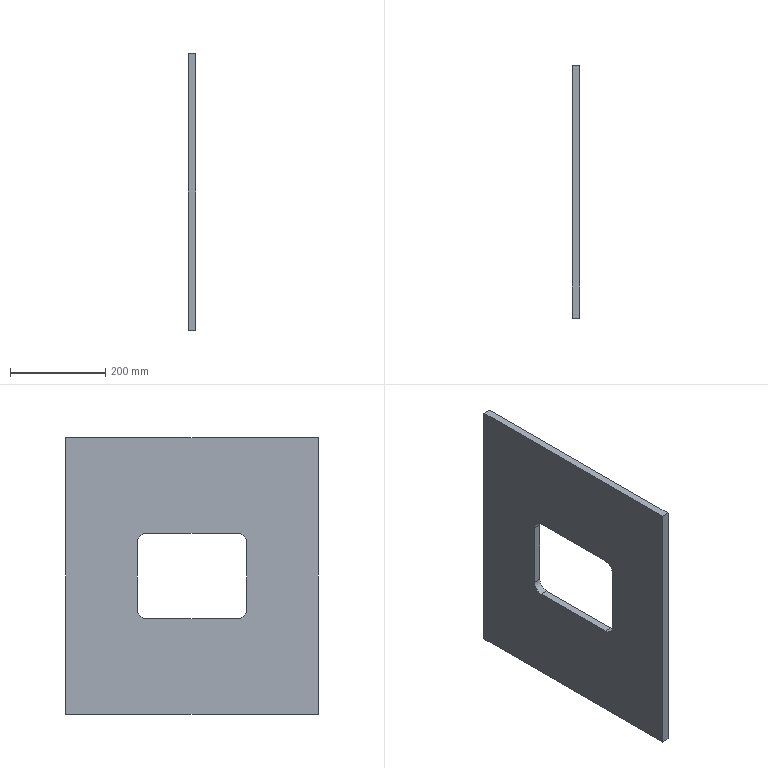Component | SolidWorks | ElectromagneticBeamRibPlate3-2 | 1 solid | 14 faces | box 16 x 530 x 580 mm | volume 4261494 mm3 | plane 10 | cylinder 4 | commonest cylinder face diameters 40 x4 | material Plain Carbon Steel
STEP:
#1=COLOUR_RGB('',0.7922,0.8196,0.9333);
#2=FILL_AREA_STYLE_COLOUR('',#1);
#3=FILL_AREA_STYLE('',(#2));
#4=SURFACE_STYLE_FILL_AREA(#3);
#5=SURFACE_SIDE_STYLE('',(#4));
#6=SURFACE_STYLE_USAGE(.BOTH.,#5);
#7=PRESENTATION_STYLE_ASSIGNMENT((#6));
#8=CARTESIAN_POINT('',(417.423,116.997,262.758));
#9=VERTEX_POINT('',#8);
#10=CARTESIAN_POINT('',(417.423,116.997,239.923));
#11=VERTEX_POINT('',#10);
#12=CARTESIAN_POINT('',(417.423,116.997,262.758));
#13=DIRECTION('',(0.,0.,-1.));
#14=VECTOR('',#13,39.37);
#15=LINE('',#12,#14);
#16=EDGE_CURVE('',#9,#11,#15,.T.);
#17=ORIENTED_EDGE('',*,*,#16,.F.);
#18=CARTESIAN_POINT('',(416.793,116.997,262.758));
#19=VERTEX_POINT('',#18);
#20=CARTESIAN_POINT('',(416.793,116.997,262.758));
#21=DIRECTION('',(1.,-0.,0.));
#22=VECTOR('',#21,39.37);
#23=LINE('',#20,#22);
#24=EDGE_CURVE('',#19,#9,#23,.T.);
#25=ORIENTED_EDGE('',*,*,#24,.F.);
#26=CARTESIAN_POINT('',(416.793,116.997,239.923));
#27=VERTEX_POINT('',#26);
#28=CARTESIAN_POINT('',(416.793,116.997,262.758));
#29=DIRECTION('',(0.,0.,-1.));
#30=VECTOR('',#29,39.37);
#31=LINE('',#28,#30);
#32=EDGE_CURVE('',#19,#27,#31,.T.);
#33=ORIENTED_EDGE('',*,*,#32,.T.);
#34=CARTESIAN_POINT('',(416.793,116.997,239.923));
#35=DIRECTION('',(1.,-0.,0.));
#36=VECTOR('',#35,39.37);
#37=LINE('',#34,#36);
#38=EDGE_CURVE('',#27,#11,#37,.T.);
#39=ORIENTED_EDGE('',*,*,#38,.T.);
#40=EDGE_LOOP('',(#17,#25,#33,#39));
#41=FACE_OUTER_BOUND('',#40,.T.);
#42=CARTESIAN_POINT('',(416.793,116.997,262.758));
#43=DIRECTION('',(-0.,-1.,-0.));
#44=DIRECTION('',(0.,0.,-1.));
#45=AXIS2_PLACEMENT_3D('',#42,#43,#44);
#46=PLANE('',#45);
#47=ADVANCED_FACE('',(#41),#46,.T.);
#48=CARTESIAN_POINT('',(417.423,137.863,262.758));
#49=VERTEX_POINT('',#48);
#50=CARTESIAN_POINT('',(417.423,116.997,262.758));
#51=DIRECTION('',(-0.,-1.,0.));
#52=VECTOR('',#51,39.37);
#53=LINE('',#50,#52);
#54=EDGE_CURVE('',#49,#9,#53,.T.);
#55=ORIENTED_EDGE('',*,*,#54,.F.);
#56=CARTESIAN_POINT('',(416.793,137.863,262.758));
#57=VERTEX_POINT('',#56);
#58=CARTESIAN_POINT('',(416.793,137.863,262.758));
#59=DIRECTION('',(1.,-0.,0.));
#60=VECTOR('',#59,39.37);
#61=LINE('',#58,#60);
#62=EDGE_CURVE('',#57,#49,#61,.T.);
#63=ORIENTED_EDGE('',*,*,#62,.F.);
#64=CARTESIAN_POINT('',(416.793,116.997,262.758));
#65=DIRECTION('',(-0.,-1.,0.));
#66=VECTOR('',#65,39.37);
#67=LINE('',#64,#66);
#68=EDGE_CURVE('',#57,#19,#67,.T.);
#69=ORIENTED_EDGE('',*,*,#68,.T.);
#70=ORIENTED_EDGE('',*,*,#24,.T.);
#71=EDGE_LOOP('',(#55,#63,#69,#70));
#72=FACE_OUTER_BOUND('',#71,.T.);
#73=CARTESIAN_POINT('',(416.793,116.997,262.758));
#74=DIRECTION('',(0.,0.,1.));
#75=DIRECTION('',(-0.,-1.,0.));
#76=AXIS2_PLACEMENT_3D('',#73,#74,#75);
#77=PLANE('',#76);
#78=ADVANCED_FACE('',(#72),#77,.T.);
#79=CARTESIAN_POINT('',(417.423,137.863,239.923));
#80=VERTEX_POINT('',#79);
#81=CARTESIAN_POINT('',(417.423,137.863,262.758));
#82=DIRECTION('',(-0.,-0.,1.));
#83=VECTOR('',#82,39.37);
#84=LINE('',#81,#83);
#85=EDGE_CURVE('',#80,#49,#84,.T.);
#86=ORIENTED_EDGE('',*,*,#85,.F.);
#87=CARTESIAN_POINT('',(416.793,137.863,239.923));
#88=VERTEX_POINT('',#87);
#89=CARTESIAN_POINT('',(416.793,137.863,239.923));
#90=DIRECTION('',(1.,-0.,0.));
#91=VECTOR('',#90,39.37);
#92=LINE('',#89,#91);
#93=EDGE_CURVE('',#88,#80,#92,.T.);
#94=ORIENTED_EDGE('',*,*,#93,.F.);
#95=CARTESIAN_POINT('',(416.793,137.863,262.758));
#96=DIRECTION('',(-0.,-0.,1.));
#97=VECTOR('',#96,39.37);
#98=LINE('',#95,#97);
#99=EDGE_CURVE('',#88,#57,#98,.T.);
#100=ORIENTED_EDGE('',*,*,#99,.T.);
#101=ORIENTED_EDGE('',*,*,#62,.T.);
#102=EDGE_LOOP('',(#86,#94,#100,#101));
#103=FACE_OUTER_BOUND('',#102,.T.);
#104=CARTESIAN_POINT('',(416.793,137.863,262.758));
#105=DIRECTION('',(0.,1.,0.));
#106=DIRECTION('',(-0.,-0.,1.));
#107=AXIS2_PLACEMENT_3D('',#104,#105,#106);
#108=PLANE('',#107);
#109=ADVANCED_FACE('',(#103),#108,.T.);
#110=CARTESIAN_POINT('',(417.423,116.997,239.923));
#111=DIRECTION('',(0.,1.,0.));
#112=VECTOR('',#111,39.37);
#113=LINE('',#110,#112);
#114=EDGE_CURVE('',#11,#80,#113,.T.);
#115=ORIENTED_EDGE('',*,*,#114,.F.);
#116=ORIENTED_EDGE('',*,*,#38,.F.);
#117=CARTESIAN_POINT('',(416.793,116.997,239.923));
#118=DIRECTION('',(0.,1.,0.));
#119=VECTOR('',#118,39.37);
#120=LINE('',#117,#119);
#121=EDGE_CURVE('',#27,#88,#120,.T.);
#122=ORIENTED_EDGE('',*,*,#121,.T.);
#123=ORIENTED_EDGE('',*,*,#93,.T.);
#124=EDGE_LOOP('',(#115,#116,#122,#123));
#125=FACE_OUTER_BOUND('',#124,.T.);
#126=CARTESIAN_POINT('',(416.793,116.997,239.923));
#127=DIRECTION('',(0.,0.,-1.));
#128=DIRECTION('',(0.,1.,0.));
#129=AXIS2_PLACEMENT_3D('',#126,#127,#128);
#130=PLANE('',#129);
#131=ADVANCED_FACE('',(#125),#130,.T.);
#132=CARTESIAN_POINT('',(416.793,131.958,248.584));
#133=VERTEX_POINT('',#132);
#134=CARTESIAN_POINT('',(416.793,131.958,254.096));
#135=VERTEX_POINT('',#134);
#136=CARTESIAN_POINT('',(416.793,131.958,254.096));
#137=DIRECTION('',(-0.,-0.,1.));
#138=VECTOR('',#137,39.37);
#139=LINE('',#136,#138);
#140=EDGE_CURVE('',#133,#135,#139,.T.);
#141=ORIENTED_EDGE('',*,*,#140,.T.);
#142=CARTESIAN_POINT('',(416.793,131.171,254.884));
#143=VERTEX_POINT('',#142);
#144=CARTESIAN_POINT('',(416.793,131.171,254.096));
#145=DIRECTION('',(1.,-0.,0.));
#146=DIRECTION('',(0.,0.,1.));
#147=AXIS2_PLACEMENT_3D('',#144,#145,#146);
#148=CIRCLE('',#147,0.7874);
#149=EDGE_CURVE('',#135,#143,#148,.T.);
#150=ORIENTED_EDGE('',*,*,#149,.T.);
#151=CARTESIAN_POINT('',(416.793,123.69,254.884));
#152=VERTEX_POINT('',#151);
#153=CARTESIAN_POINT('',(416.793,123.69,254.884));
#154=DIRECTION('',(-0.,-1.,0.));
#155=VECTOR('',#154,39.37);
#156=LINE('',#153,#155);
#157=EDGE_CURVE('',#143,#152,#156,.T.);
#158=ORIENTED_EDGE('',*,*,#157,.T.);
#159=CARTESIAN_POINT('',(416.793,122.903,254.096));
#160=VERTEX_POINT('',#159);
#161=CARTESIAN_POINT('',(416.793,123.69,254.096));
#162=DIRECTION('',(1.,-0.,0.));
#163=DIRECTION('',(0.,0.,-1.));
#164=AXIS2_PLACEMENT_3D('',#161,#162,#163);
#165=CIRCLE('',#164,0.7874);
#166=EDGE_CURVE('',#152,#160,#165,.T.);
#167=ORIENTED_EDGE('',*,*,#166,.T.);
#168=CARTESIAN_POINT('',(416.793,122.903,248.584));
#169=VERTEX_POINT('',#168);
#170=CARTESIAN_POINT('',(416.793,122.903,254.096));
#171=DIRECTION('',(0.,0.,-1.));
#172=VECTOR('',#171,39.37);
#173=LINE('',#170,#172);
#174=EDGE_CURVE('',#160,#169,#173,.T.);
#175=ORIENTED_EDGE('',*,*,#174,.T.);
#176=CARTESIAN_POINT('',(416.793,123.69,247.797));
#177=VERTEX_POINT('',#176);
#178=CARTESIAN_POINT('',(416.793,123.69,248.584));
#179=DIRECTION('',(1.,-0.,0.));
#180=DIRECTION('',(0.,0.,-1.));
#181=AXIS2_PLACEMENT_3D('',#178,#179,#180);
#182=CIRCLE('',#181,0.7874);
#183=EDGE_CURVE('',#169,#177,#182,.T.);
#184=ORIENTED_EDGE('',*,*,#183,.T.);
#185=CARTESIAN_POINT('',(416.793,131.171,247.797));
#186=VERTEX_POINT('',#185);
#187=CARTESIAN_POINT('',(416.793,123.69,247.797));
#188=DIRECTION('',(0.,1.,0.));
#189=VECTOR('',#188,39.37);
#190=LINE('',#187,#189);
#191=EDGE_CURVE('',#177,#186,#190,.T.);
#192=ORIENTED_EDGE('',*,*,#191,.T.);
#193=CARTESIAN_POINT('',(416.793,131.171,248.584));
#194=DIRECTION('',(1.,-0.,0.));
#195=DIRECTION('',(0.,0.,-1.));
#196=AXIS2_PLACEMENT_3D('',#193,#194,#195);
#197=CIRCLE('',#196,0.7874);
#198=EDGE_CURVE('',#186,#133,#197,.T.);
#199=ORIENTED_EDGE('',*,*,#198,.T.);
#200=EDGE_LOOP('',(#141,#150,#158,#167,#175,#184,#192,#199));
#201=FACE_BOUND('',#200,.T.);
#202=ORIENTED_EDGE('',*,*,#32,.F.);
#203=ORIENTED_EDGE('',*,*,#68,.F.);
#204=ORIENTED_EDGE('',*,*,#99,.F.);
#205=ORIENTED_EDGE('',*,*,#121,.F.);
#206=EDGE_LOOP('',(#202,#203,#204,#205));
#207=FACE_OUTER_BOUND('',#206,.T.);
#208=CARTESIAN_POINT('',(416.793,116.997,262.758));
#209=DIRECTION('',(1.,-0.,0.));
#210=DIRECTION('',(0.,0.,-1.));
#211=AXIS2_PLACEMENT_3D('',#208,#209,#210);
#212=PLANE('',#211);
#213=ADVANCED_FACE('',(#201,#207),#212,.F.);
#214=CARTESIAN_POINT('',(417.423,131.958,254.096));
#215=VERTEX_POINT('',#214);
#216=CARTESIAN_POINT('',(417.423,131.171,254.884));
#217=VERTEX_POINT('',#216);
#218=CARTESIAN_POINT('',(417.423,131.171,254.096));
#219=DIRECTION('',(1.,-0.,0.));
#220=DIRECTION('',(0.,0.,1.));
#221=AXIS2_PLACEMENT_3D('',#218,#219,#220);
#222=CIRCLE('',#221,0.7874);
#223=EDGE_CURVE('',#215,#217,#222,.T.);
#224=ORIENTED_EDGE('',*,*,#223,.F.);
#225=CARTESIAN_POINT('',(417.423,131.958,248.584));
#226=VERTEX_POINT('',#225);
#227=CARTESIAN_POINT('',(417.423,131.958,254.096));
#228=DIRECTION('',(-0.,-0.,1.));
#229=VECTOR('',#228,39.37);
#230=LINE('',#227,#229);
#231=EDGE_CURVE('',#226,#215,#230,.T.);
#232=ORIENTED_EDGE('',*,*,#231,.F.);
#233=CARTESIAN_POINT('',(417.423,131.171,247.797));
#234=VERTEX_POINT('',#233);
#235=CARTESIAN_POINT('',(417.423,131.171,248.584));
#236=DIRECTION('',(1.,-0.,0.));
#237=DIRECTION('',(0.,0.,-1.));
#238=AXIS2_PLACEMENT_3D('',#235,#236,#237);
#239=CIRCLE('',#238,0.7874);
#240=EDGE_CURVE('',#234,#226,#239,.T.);
#241=ORIENTED_EDGE('',*,*,#240,.F.);
#242=CARTESIAN_POINT('',(417.423,123.69,247.797));
#243=VERTEX_POINT('',#242);
#244=CARTESIAN_POINT('',(417.423,123.69,247.797));
#245=DIRECTION('',(0.,1.,0.));
#246=VECTOR('',#245,39.37);
#247=LINE('',#244,#246);
#248=EDGE_CURVE('',#243,#234,#247,.T.);
#249=ORIENTED_EDGE('',*,*,#248,.F.);
#250=CARTESIAN_POINT('',(417.423,122.903,248.584));
#251=VERTEX_POINT('',#250);
#252=CARTESIAN_POINT('',(417.423,123.69,248.584));
#253=DIRECTION('',(1.,-0.,0.));
#254=DIRECTION('',(0.,0.,-1.));
#255=AXIS2_PLACEMENT_3D('',#252,#253,#254);
#256=CIRCLE('',#255,0.7874);
#257=EDGE_CURVE('',#251,#243,#256,.T.);
#258=ORIENTED_EDGE('',*,*,#257,.F.);
#259=CARTESIAN_POINT('',(417.423,122.903,254.096));
#260=VERTEX_POINT('',#259);
#261=CARTESIAN_POINT('',(417.423,122.903,254.096));
#262=DIRECTION('',(0.,0.,-1.));
#263=VECTOR('',#262,39.37);
#264=LINE('',#261,#263);
#265=EDGE_CURVE('',#260,#251,#264,.T.);
#266=ORIENTED_EDGE('',*,*,#265,.F.);
#267=CARTESIAN_POINT('',(417.423,123.69,254.884));
#268=VERTEX_POINT('',#267);
#269=CARTESIAN_POINT('',(417.423,123.69,254.096));
#270=DIRECTION('',(1.,-0.,0.));
#271=DIRECTION('',(0.,0.,-1.));
#272=AXIS2_PLACEMENT_3D('',#269,#270,#271);
#273=CIRCLE('',#272,0.7874);
#274=EDGE_CURVE('',#268,#260,#273,.T.);
#275=ORIENTED_EDGE('',*,*,#274,.F.);
#276=CARTESIAN_POINT('',(417.423,123.69,254.884));
#277=DIRECTION('',(-0.,-1.,0.));
#278=VECTOR('',#277,39.37);
#279=LINE('',#276,#278);
#280=EDGE_CURVE('',#217,#268,#279,.T.);
#281=ORIENTED_EDGE('',*,*,#280,.F.);
#282=EDGE_LOOP('',(#224,#232,#241,#249,#258,#266,#275,#281));
#283=FACE_BOUND('',#282,.T.);
#284=ORIENTED_EDGE('',*,*,#16,.T.);
#285=ORIENTED_EDGE('',*,*,#114,.T.);
#286=ORIENTED_EDGE('',*,*,#85,.T.);
#287=ORIENTED_EDGE('',*,*,#54,.T.);
#288=EDGE_LOOP('',(#284,#285,#286,#287));
#289=FACE_OUTER_BOUND('',#288,.T.);
#290=CARTESIAN_POINT('',(417.423,116.997,262.758));
#291=DIRECTION('',(1.,-0.,0.));
#292=DIRECTION('',(0.,0.,-1.));
#293=AXIS2_PLACEMENT_3D('',#290,#291,#292);
#294=PLANE('',#293);
#295=ADVANCED_FACE('',(#283,#289),#294,.T.);
#296=ORIENTED_EDGE('',*,*,#223,.T.);
#297=CARTESIAN_POINT('',(416.793,131.171,254.884));
#298=DIRECTION('',(1.,-0.,0.));
#299=VECTOR('',#298,39.37);
#300=LINE('',#297,#299);
#301=EDGE_CURVE('',#143,#217,#300,.T.);
#302=ORIENTED_EDGE('',*,*,#301,.F.);
#303=ORIENTED_EDGE('',*,*,#149,.F.);
#304=CARTESIAN_POINT('',(416.793,131.958,254.096));
#305=DIRECTION('',(1.,-0.,0.));
#306=VECTOR('',#305,39.37);
#307=LINE('',#304,#306);
#308=EDGE_CURVE('',#135,#215,#307,.T.);
#309=ORIENTED_EDGE('',*,*,#308,.T.);
#310=EDGE_LOOP('',(#296,#302,#303,#309));
#311=FACE_OUTER_BOUND('',#310,.T.);
#312=CARTESIAN_POINT('',(416.793,131.171,254.096));
#313=DIRECTION('',(1.,-0.,0.));
#314=DIRECTION('',(0.,0.,-1.));
#315=AXIS2_PLACEMENT_3D('',#312,#313,#314);
#316=CYLINDRICAL_SURFACE('',#315,0.7874);
#317=ADVANCED_FACE('',(#311),#316,.F.);
#318=ORIENTED_EDGE('',*,*,#231,.T.);
#319=ORIENTED_EDGE('',*,*,#308,.F.);
#320=ORIENTED_EDGE('',*,*,#140,.F.);
#321=CARTESIAN_POINT('',(416.793,131.958,248.584));
#322=DIRECTION('',(1.,-0.,0.));
#323=VECTOR('',#322,39.37);
#324=LINE('',#321,#323);
#325=EDGE_CURVE('',#133,#226,#324,.T.);
#326=ORIENTED_EDGE('',*,*,#325,.T.);
#327=EDGE_LOOP('',(#318,#319,#320,#326));
#328=FACE_OUTER_BOUND('',#327,.T.);
#329=CARTESIAN_POINT('',(416.793,131.958,254.096));
#330=DIRECTION('',(0.,1.,0.));
#331=DIRECTION('',(-0.,-0.,1.));
#332=AXIS2_PLACEMENT_3D('',#329,#330,#331);
#333=PLANE('',#332);
#334=ADVANCED_FACE('',(#328),#333,.F.);
#335=ORIENTED_EDGE('',*,*,#240,.T.);
#336=ORIENTED_EDGE('',*,*,#325,.F.);
#337=ORIENTED_EDGE('',*,*,#198,.F.);
#338=CARTESIAN_POINT('',(416.793,131.171,247.797));
#339=DIRECTION('',(1.,-0.,0.));
#340=VECTOR('',#339,39.37);
#341=LINE('',#338,#340);
#342=EDGE_CURVE('',#186,#234,#341,.T.);
#343=ORIENTED_EDGE('',*,*,#342,.T.);
#344=EDGE_LOOP('',(#335,#336,#337,#343));
#345=FACE_OUTER_BOUND('',#344,.T.);
#346=CARTESIAN_POINT('',(416.793,131.171,248.584));
#347=DIRECTION('',(1.,-0.,0.));
#348=DIRECTION('',(0.,0.,-1.));
#349=AXIS2_PLACEMENT_3D('',#346,#347,#348);
#350=CYLINDRICAL_SURFACE('',#349,0.7874);
#351=ADVANCED_FACE('',(#345),#350,.F.);
#352=ORIENTED_EDGE('',*,*,#248,.T.);
#353=ORIENTED_EDGE('',*,*,#342,.F.);
#354=ORIENTED_EDGE('',*,*,#191,.F.);
#355=CARTESIAN_POINT('',(416.793,123.69,247.797));
#356=DIRECTION('',(1.,-0.,0.));
#357=VECTOR('',#356,39.37);
#358=LINE('',#355,#357);
#359=EDGE_CURVE('',#177,#243,#358,.T.);
#360=ORIENTED_EDGE('',*,*,#359,.T.);
#361=EDGE_LOOP('',(#352,#353,#354,#360));
#362=FACE_OUTER_BOUND('',#361,.T.);
#363=CARTESIAN_POINT('',(416.793,123.69,247.797));
#364=DIRECTION('',(0.,0.,-1.));
#365=DIRECTION('',(0.,1.,0.));
#366=AXIS2_PLACEMENT_3D('',#363,#364,#365);
#367=PLANE('',#366);
#368=ADVANCED_FACE('',(#362),#367,.F.);
#369=ORIENTED_EDGE('',*,*,#257,.T.);
#370=ORIENTED_EDGE('',*,*,#359,.F.);
#371=ORIENTED_EDGE('',*,*,#183,.F.);
#372=CARTESIAN_POINT('',(416.793,122.903,248.584));
#373=DIRECTION('',(1.,-0.,0.));
#374=VECTOR('',#373,39.37);
#375=LINE('',#372,#374);
#376=EDGE_CURVE('',#169,#251,#375,.T.);
#377=ORIENTED_EDGE('',*,*,#376,.T.);
#378=EDGE_LOOP('',(#369,#370,#371,#377));
#379=FACE_OUTER_BOUND('',#378,.T.);
#380=CARTESIAN_POINT('',(416.793,123.69,248.584));
#381=DIRECTION('',(1.,-0.,0.));
#382=DIRECTION('',(0.,0.,-1.));
#383=AXIS2_PLACEMENT_3D('',#380,#381,#382);
#384=CYLINDRICAL_SURFACE('',#383,0.7874);
#385=ADVANCED_FACE('',(#379),#384,.F.);
#386=ORIENTED_EDGE('',*,*,#265,.T.);
#387=ORIENTED_EDGE('',*,*,#376,.F.);
#388=ORIENTED_EDGE('',*,*,#174,.F.);
#389=CARTESIAN_POINT('',(416.793,122.903,254.096));
#390=DIRECTION('',(1.,-0.,0.));
#391=VECTOR('',#390,39.37);
#392=LINE('',#389,#391);
#393=EDGE_CURVE('',#160,#260,#392,.T.);
#394=ORIENTED_EDGE('',*,*,#393,.T.);
#395=EDGE_LOOP('',(#386,#387,#388,#394));
#396=FACE_OUTER_BOUND('',#395,.T.);
#397=CARTESIAN_POINT('',(416.793,122.903,254.096));
#398=DIRECTION('',(-0.,-1.,-0.));
#399=DIRECTION('',(0.,0.,-1.));
#400=AXIS2_PLACEMENT_3D('',#397,#398,#399);
#401=PLANE('',#400);
#402=ADVANCED_FACE('',(#396),#401,.F.);
#403=ORIENTED_EDGE('',*,*,#274,.T.);
#404=ORIENTED_EDGE('',*,*,#393,.F.);
#405=ORIENTED_EDGE('',*,*,#166,.F.);
#406=CARTESIAN_POINT('',(416.793,123.69,254.884));
#407=DIRECTION('',(1.,-0.,0.));
#408=VECTOR('',#407,39.37);
#409=LINE('',#406,#408);
#410=EDGE_CURVE('',#152,#268,#409,.T.);
#411=ORIENTED_EDGE('',*,*,#410,.T.);
#412=EDGE_LOOP('',(#403,#404,#405,#411));
#413=FACE_OUTER_BOUND('',#412,.T.);
#414=CARTESIAN_POINT('',(416.793,123.69,254.096));
#415=DIRECTION('',(1.,-0.,0.));
#416=DIRECTION('',(0.,0.,-1.));
#417=AXIS2_PLACEMENT_3D('',#414,#415,#416);
#418=CYLINDRICAL_SURFACE('',#417,0.7874);
#419=ADVANCED_FACE('',(#413),#418,.F.);
#420=ORIENTED_EDGE('',*,*,#280,.T.);
#421=ORIENTED_EDGE('',*,*,#410,.F.);
#422=ORIENTED_EDGE('',*,*,#157,.F.);
#423=ORIENTED_EDGE('',*,*,#301,.T.);
#424=EDGE_LOOP('',(#420,#421,#422,#423));
#425=FACE_OUTER_BOUND('',#424,.T.);
#426=CARTESIAN_POINT('',(416.793,123.69,254.884));
#427=DIRECTION('',(0.,0.,1.));
#428=DIRECTION('',(-0.,-1.,0.));
#429=AXIS2_PLACEMENT_3D('',#426,#427,#428);
#430=PLANE('',#429);
#431=ADVANCED_FACE('',(#425),#430,.F.);
#432=CLOSED_SHELL('',(#47,#78,#109,#131,#213,#295,#317,#334,#351,#368,#385,#402,#419,#431));
#433=MANIFOLD_SOLID_BREP('',#432);
#434=STYLED_ITEM('',(#7),#433);
#435=(LENGTH_UNIT()NAMED_UNIT(*)SI_UNIT($,.METRE.));
#436=LENGTH_MEASURE_WITH_UNIT(LENGTH_MEASURE(0.0254),#435);
#437=DIMENSIONAL_EXPONENTS(1.,0.,0.,0.,0.,0.,0.);
#438=(CONVERSION_BASED_UNIT('',#436)LENGTH_UNIT()NAMED_UNIT(#437));
#439=UNCERTAINTY_MEASURE_WITH_UNIT(LENGTH_MEASURE(0.00001),#438,'','');
#440=(NAMED_UNIT(*)PLANE_ANGLE_UNIT()SI_UNIT($,.RADIAN.));
#441=(NAMED_UNIT(*)SI_UNIT($,.STERADIAN.)SOLID_ANGLE_UNIT());
#442=(GEOMETRIC_REPRESENTATION_CONTEXT(3)GLOBAL_UNCERTAINTY_ASSIGNED_CONTEXT((#439))GLOBAL_UNIT_ASSIGNED_CONTEXT((#438,#440,#441))REPRESENTATION_CONTEXT('',''));
#443=MECHANICAL_DESIGN_GEOMETRIC_PRESENTATION_REPRESENTATION('',(#434),#442);
#444=PRESENTATION_LAYER_ASSIGNMENT('','',(#434));
#445=CARTESIAN_POINT('',(0.,0.,0.));
#446=DIRECTION('',(0.,0.,1.));
#447=DIRECTION('',(1.,0.,0.));
#448=AXIS2_PLACEMENT_3D('',#445,#446,#447);
#449=(LENGTH_UNIT()NAMED_UNIT(*)SI_UNIT($,.METRE.));
#450=LENGTH_MEASURE_WITH_UNIT(LENGTH_MEASURE(0.0254),#449);
#451=DIMENSIONAL_EXPONENTS(1.,0.,0.,0.,0.,0.,0.);
#452=(CONVERSION_BASED_UNIT('',#450)LENGTH_UNIT()NAMED_UNIT(#451));
#453=UNCERTAINTY_MEASURE_WITH_UNIT(LENGTH_MEASURE(0.00001),#452,'','');
#454=(NAMED_UNIT(*)PLANE_ANGLE_UNIT()SI_UNIT($,.RADIAN.));
#455=(NAMED_UNIT(*)SI_UNIT($,.STERADIAN.)SOLID_ANGLE_UNIT());
#456=(GEOMETRIC_REPRESENTATION_CONTEXT(3)GLOBAL_UNCERTAINTY_ASSIGNED_CONTEXT((#453))GLOBAL_UNIT_ASSIGNED_CONTEXT((#452,#454,#455))REPRESENTATION_CONTEXT('',''));
#457=ADVANCED_BREP_SHAPE_REPRESENTATION('',(#433,#448),#456);